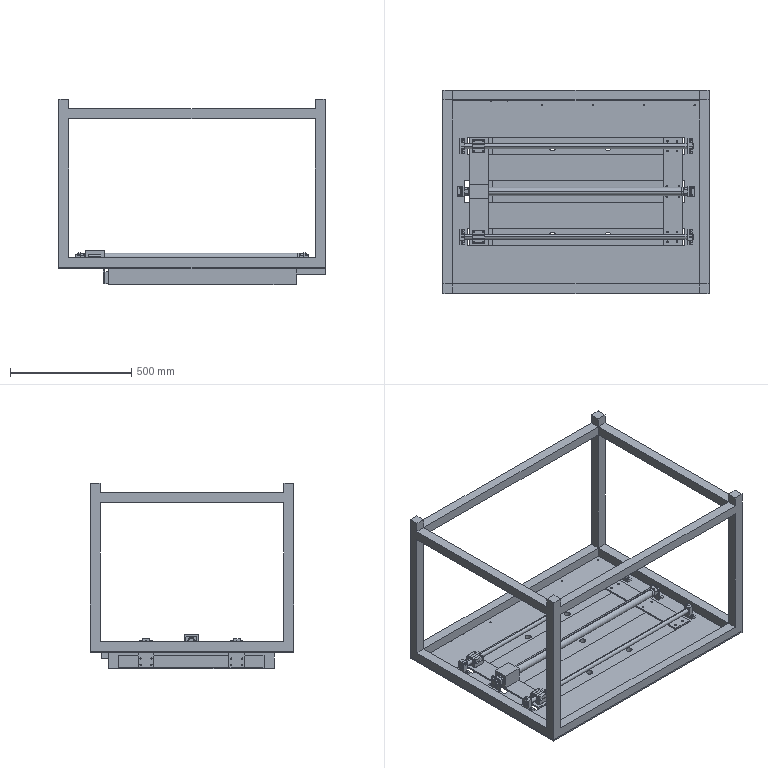Assembly | SolidWorks | mm | 23 component files | 23 solids | 758 faces | box 1100 x 840 x 766 mm | volume 57780963 mm3 | cylinder 350 | plane 326 | cone 58 | spline 24 | commonest cylinder face diameters 5 x60 6.5 x56 6.6 x40 11 x24 1 x24 20 x20 4.917 x16 32 x12
Bill of materials:
DC-Motor-110 | 1 |  | Open rectangular box frame made of straight square-section bars: a top and a bottom rectangular ring of rails joined by four vertical corner posts. The posts stick up slightly above the top rails.
DC-Motor-111 | 1 |  | Thin flat rectangular plate with three long parallel rectangular slots. Small round holes sit beside the slot ends and run in a row along one long edge.
DC-Motor-112 | 1 |  | Long straight bar with a rectangular, near-square section. Four small round holes are evenly spaced along one face.
DC-Motor-113 | 2 |  | L-shaped angle bracket. The upright leg has chamfered top corners, one large round hole and one smaller round hole below it. The shorter base leg has two round holes.
DC-Motor-114 | 2 |  | Plain, long, solid cylindrical rod of uniform diameter with flat ends.
DC-Motor-115 | 2 |  | Long, thin, flat rectangular plate with twelve small round holes in three groups of four: one group near each end and one in the middle. The middle group is spaced slightly wider.
DC-Motor-116 | 2 |  | L-shaped angle bracket of uniform thickness. One leg has two larger round holes; the other, longer leg has four smaller round holes in a rectangular pattern.
DC-Motor-117 | 1 |  | Long, flat rectangular bar standing on its edge, with two groups of four small round holes (2x2 pattern) near each end, drilled through the broad face.
GFF01-D20 | 4 |  | T-shaped block with an upright body and a wider base flange that has one round hole on each side. The upright has a large horizontal round bore and a narrow slit from the top down into the bore. A cross hole holds a socket-head screw that spans the slit.
LMW01-d20 | 2 |  | Rectangular housing block with a large central horizontal through bore that has a stepped or recessed entry. The top has a raised ridge with chamfered flanks. There are four round holes near the top corners, chamfered lower side edges with a longitudinal groove, and a shallow recess on the underside.
RMS32X50_Body | 1 |  | Plain rectangular block with one large round hole through the centre of one face pair. Concentric rings at the hole entry suggest a chamfer, groove, or counterbore.
RMS32X50_Nut | 2 |  | Thin hexagonal ring with a large round central bore and chamfered outer corners on both faces. The proportions resemble a thin hex nut.
RMS32X800(0)-fcv | 1 |  | Long, slender straight rod. The main body has a faceted (polygonal) cross-section, and each end steps down to a short shoulder and then a smaller round end pin. Both ends look the same.
Tray | 1 |  | Flat rectangular plate of even thickness, nearly square, with five small round holes: four at the corners of a rectangle and one in the middle, all centred on the plate.
Mates:
1. coincident | DC-Motor-110-1 face at (2.208, 11.801, -420) dir (0, 0, -1) | DC-Motor-111-1 face at (2.208, 11.801, -420) dir (0, 0, 1)
2. coincident | DC-Motor-110-1 face at (552.208, -408.199, -380) dir (1, 0, 0) | DC-Motor-111-1 face at (552.208, -408.199, -420) dir (1, 0, 0)
3. coincident | DC-Motor-110-1 face at (552.208, 431.801, -380) dir (0, 1, 0) | DC-Motor-111-1 face at (552.208, 431.801, -420) dir (0, 1, 0)
4. coincident | DC-Motor-111-1 face at (2.208, 11.801, -426) dir (0, 0, -1) | Tray-1 face at (44.708, 14.301, -426) dir (0, 0, 1)
5. coincident | DC-Motor-111-1 face at (2.208, 11.801, -426) dir (0, 0, -1) | DC-Motor-112-1 face at (177.208, 371.801, -426) dir (0, 0, 1)
6. coincident | Tray-1 face at (432.208, 356.801, -426) dir (0, 1, 0) | DC-Motor-112-1 face at (-197.792, 356.801, -451) dir (0, -1, 0)
7. coincident | DC-Motor-110-1 face at (552.208, -408.199, -380) dir (1, 0, 0) | DC-Motor-112-1 face at (552.208, 356.801, -451) dir (1, 0, 0)
8. distance | DC-Motor-110-1 face at (552.208, 431.801, -380) dir (0, 1, 0) | Tray-1 face at (432.208, 356.801, -426) dir (0, 1, 0)
9. width | RMS32X800_0-1/RMS32X50_Body-1 face at (-357.792, 44.301, -410) dir (0, 1, 0) | RMS32X800_0-1/RMS32X50_Body-1 face at (-357.792, -15.699, -350) dir (0, -1, 0) | Tray-1 face at (432.208, -328.199, -426) dir (0, -1, 0) | Tray-1 face at (432.208, 356.801, -426) dir (0, 1, 0)
10. parallel | DC-Motor-111-1 face at (2.208, 11.801, -420) dir (0, 0, 1) | RMS32X800_0-1/RMS32X50_Body-1 face at (-357.792, 44.301, -350) dir (0, 0, 1)
11. width | RMS32X800_0-1/RMS32X800(0)-fcv-1 face at (480.208, 2.221, -380) dir (1, 0, 0) | RMS32X800_0-1/RMS32X800(0)-fcv-1 face at (-475.792, 14.301, -380) dir (-1, 0, 0) | DC-Motor-110-1 face at (-547.792, -408.199, -380) dir (-1, 0, 0) | DC-Motor-110-1 face at (552.208, -408.199, -380) dir (1, 0, 0)
12. concentric | RMS32X800_0-1/RMS32X800(0)-fcv-1 face at (-433.792, 14.301, -380) dir (-1, 0, 0) r 13 | DC-Motor-113-1 face at (-422.792, 14.301, -380) dir (-1, 0, 0) r 13.25
13. coincident | RMS32X800_0-1/RMS32X800(0)-fcv-1 face at (-459.792, 1.301, -380) dir (-1, 0, 0) | DC-Motor-113-1 face at (-459.792, 36.801, -360) dir (1, 0, 0)
14. parallel | RMS32X800_0-1/RMS32X50_Body-1 face at (-357.792, -15.699, -350) dir (0, -1, 0) | DC-Motor-113-1 face at (-459.792, -8.199, -420) dir (0, -1, 0)
15. coincident | DC-Motor-111-1 face at (2.208, 11.801, -420) dir (0, 0, 1) | DC-Motor-113-1 face at (-459.792, 36.801, -420) dir (0, 0, -1)
16. concentric | RMS32X800_0-1/RMS32X800(0)-fcv-1 face at (480.208, 14.301, -380) dir (-1, 0, 0) r 13 | DC-Motor-113-2 face at (427.208, 14.301, -380) dir (1, 0, 0) r 13.25
17. coincident | DC-Motor-111-1 face at (2.208, 11.801, -420) dir (0, 0, 1) | DC-Motor-113-2 face at (464.208, -8.199, -420) dir (0, 0, -1)
18. coincident | RMS32X800_0-1/RMS32X800(0)-fcv-1 face at (464.208, -4.949, -380) dir (1, 0, 0) | DC-Motor-113-2 face at (464.208, -8.199, -360) dir (-1, 0, 0)
19. coincident | DC-Motor-111-1 face at (2.208, 11.801, -420) dir (0, 0, 1) | GFF01-D20-1 face at (-457.792, 171.801, -420) dir (0, 0, -1)
20. parallel | RMS32X800_0-1/RMS32X50_Body-1 face at (-357.792, 44.301, -410) dir (0, 1, 0) | GFF01-D20-1 face at (-457.792, 186.801, -369.5) dir (0, -1, 0)
21. coincident | DC-Motor-111-1 face at (-457.792, -31.699, 48) dir (1, 0, 0) | GFF01-D20-1 face at (-457.792, 172.301, -410.5) dir (1, 0, 0)
22. coincident | DC-Motor-113-2 face at (464.208, -8.199, -360) dir (-1, 0, 0) | GFF01-D20-2 face at (464.208, 172.301, -410.5) dir (-1, 0, 0)
23. concentric | GFF01-D20-1 face at (-457.792, 201.801, -389) dir (1, 0, 0) r 10 | GFF01-D20-2 face at (484.208, 201.801, -389) dir (1, 0, 0) r 10
24. concentric | GFF01-D20-1 face at (-457.792, 201.801, -389) dir (1, 0, 0) r 10 | DC-Motor-114-1 face at (485.708, 201.801, -389) dir (-1, 0, 0) r 10
25. width | DC-Motor-114-1 face at (485.708, 201.801, -389) dir (1, 0, 0) | DC-Motor-114-1 face at (-479.292, 201.801, -389) dir (-1, 0, 0) | GFF01-D20-1 face at (-477.792, 172.301, -410.5) dir (-1, 0, 0) | GFF01-D20-2 face at (484.208, 172.301, -410.5) dir (1, 0, 0)
26. concentric | DC-Motor-114-1 face at (485.708, 201.801, -389) dir (-1, 0, 0) r 10 | LMW01-d20-1 face at (-425.007, 201.801, -389) dir (1, 0, 0) r 10
27. parallel | RMS32X800_0-1/RMS32X50_Body-1 face at (-357.792, 44.301, -350) dir (0, 0, 1) | LMW01-d20-1 face at (-425.007, 212.301, -410) dir (0, 0, -1)
28. distance | GFF01-D20-3 face at (-477.792, -158.199, -369.5) dir (0, 1, 0) | DC-Motor-113-1 face at (-459.792, -8.199, -420) dir (0, -1, 0)
29. coincident | RMS32X800_0-1/RMS32X50_Body-1 face at (-357.792, -15.699, -410) dir (0, 0, -1) | DC-Motor-115-1 face at (-397.792, 14.301, -410) dir (0, 0, 1)
30. width | DC-Motor-115-1 face at (-437.792, -210.699, -410) dir (-1, 0, 0) | DC-Motor-115-1 face at (-357.792, -210.699, -410) dir (1, 0, 0) | RMS32X800_0-1/RMS32X50_Body-1 face at (-357.792, 14.301, -380) dir (1, 0, 0) | RMS32X800_0-1/RMS32X50_Body-1 face at (-437.792, 14.301, -380) dir (-1, 0, 0)
31. width | DC-Motor-115-1 face at (-437.792, -210.699, -410) dir (0, -1, 0) | DC-Motor-115-1 face at (-437.792, 239.301, -410) dir (0, 1, 0) | LMW01-d20-1 face at (-425.007, 228.801, -408) dir (0, 1, 0) | LMW01-d20-2 face at (-375.007, -200.199, -408) dir (0, -1, 0)
32. coincident | DC-Motor-115-1 face at (-397.792, 14.301, -416) dir (0, 0, -1) | DC-Motor-116-1 face at (-397.792, -140.699, -416) dir (0, 0, 1)
33. width | DC-Motor-116-1 face at (-357.792, -205.699, -416) dir (0, -1, 0) | DC-Motor-116-1 face at (-357.792, -140.699, -416) dir (0, 1, 0) | DC-Motor-111-1 face at (-447.792, -209.199, -1115) dir (0, 1, 0) | DC-Motor-111-1 face at (-447.792, -137.199, -1115) dir (0, -1, 0)
34. coincident | DC-Motor-115-1 face at (-357.792, -210.699, -410) dir (1, 0, 0) | DC-Motor-116-1 face at (-357.792, -140.699, -416) dir (1, 0, 0)
35. coincident | DC-Motor-116-1 face at (-397.792, -140.699, -422) dir (0, 0, -1) | DC-Motor-116-2 face at (-397.792, 234.301, -422) dir (0, 0, -1)
36. width | DC-Motor-116-2 face at (-357.792, 169.301, -416) dir (0, -1, 0) | DC-Motor-116-2 face at (-357.792, 234.301, -416) dir (0, 1, 0) | DC-Motor-111-1 face at (-447.792, 165.801, -1115) dir (0, 1, 0) | DC-Motor-111-1 face at (-447.792, 237.801, -1115) dir (0, -1, 0)
37. coincident | DC-Motor-116-2 face at (-357.792, 234.301, -416) dir (1, 0, 0) | DC-Motor-117-1 face at (-357.792, 14.301, -463) dir (-1, 0, 0)
38. coincident | DC-Motor-116-2 face at (-363.792, 234.301, -488) dir (0, 0, -1) | DC-Motor-117-1 face at (-357.792, -285.699, -488) dir (0, 0, -1)
39. width | DC-Motor-117-1 face at (-357.792, -285.699, -438) dir (0, -1, 0) | DC-Motor-117-1 face at (-357.792, 314.301, -438) dir (0, 1, 0) | DC-Motor-116-2 face at (-357.792, 234.301, -416) dir (0, 1, 0) | DC-Motor-116-1 face at (-357.792, -205.699, -416) dir (0, -1, 0)
40. coincident | DC-Motor-116-1 face at (-357.792, -140.699, -416) dir (1, 0, 0) | DC-Motor-117-1 face at (-357.792, 14.301, -463) dir (-1, 0, 0)
41. coincident | Tray-1 face at (-342.792, -328.199, -426) dir (-1, 0, 0) | DC-Motor-117-1 face at (-342.792, 14.301, -463) dir (1, 0, 0)